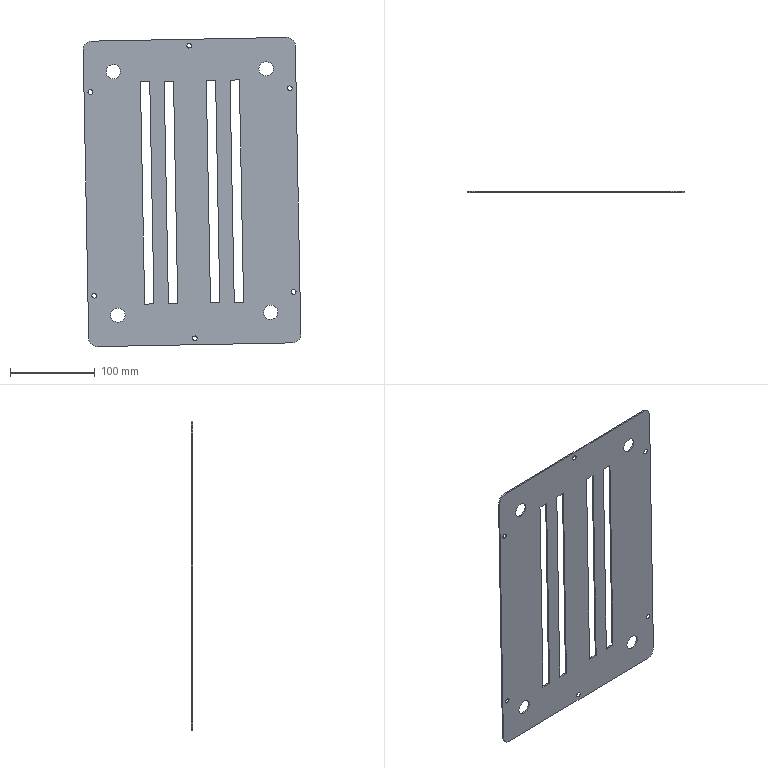Component | SolidWorks | 16MeshPlateOneOutOfTwo-1 | 1 solid | 46 faces | volume 115856 mm3 | plane 22 | cone 12 | cylinder 12 | commonest cylinder face diameters 17 x8 20 x4 | material A3 Steel